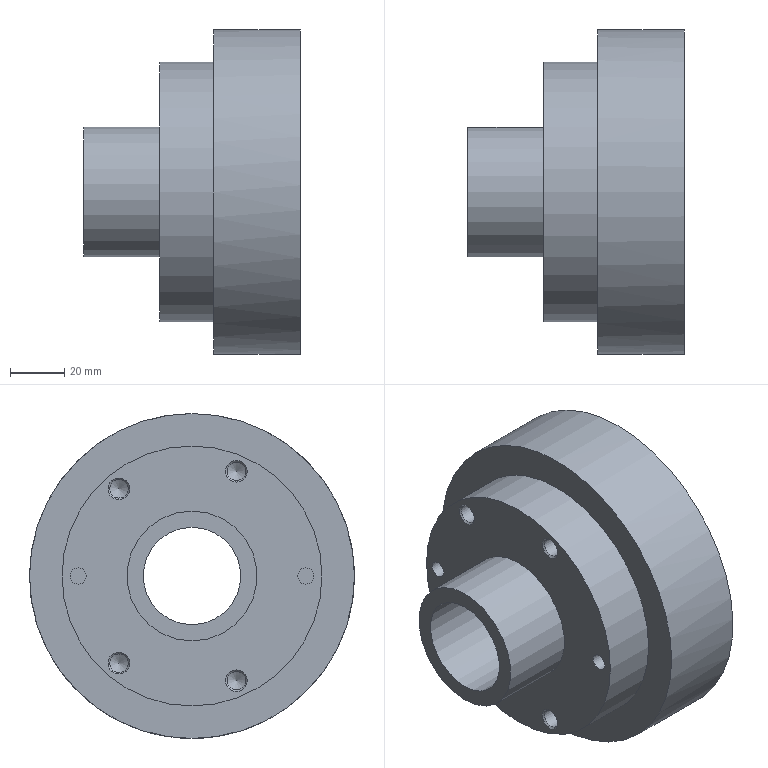Component | NX | VOLUTE_CASING | 1 solid | 45 faces | volume 319826 mm3 | cone 18 | cylinder 17 | plane 10 | commonest cylinder face diameters 5 x4 6 x4 6.8 x4 96 x2 120 x1 48 x1 36 x1